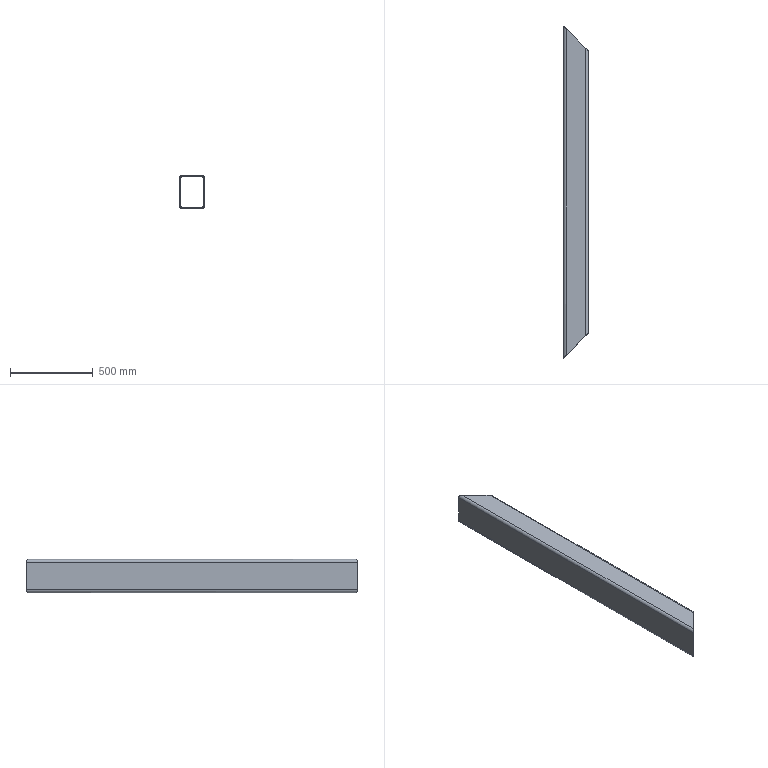Component | NX | AAAAAAAAAAAAAAAAAAAAAAAAAAAAAAAAAAAAAAAAAAAAAAAAAAAAAAAAAAA_14 | 1 solid | 18 faces | volume 9581494 mm3 | plane 10 | cylinder 8 | commonest cylinder face diameters 32 x4 16 x4